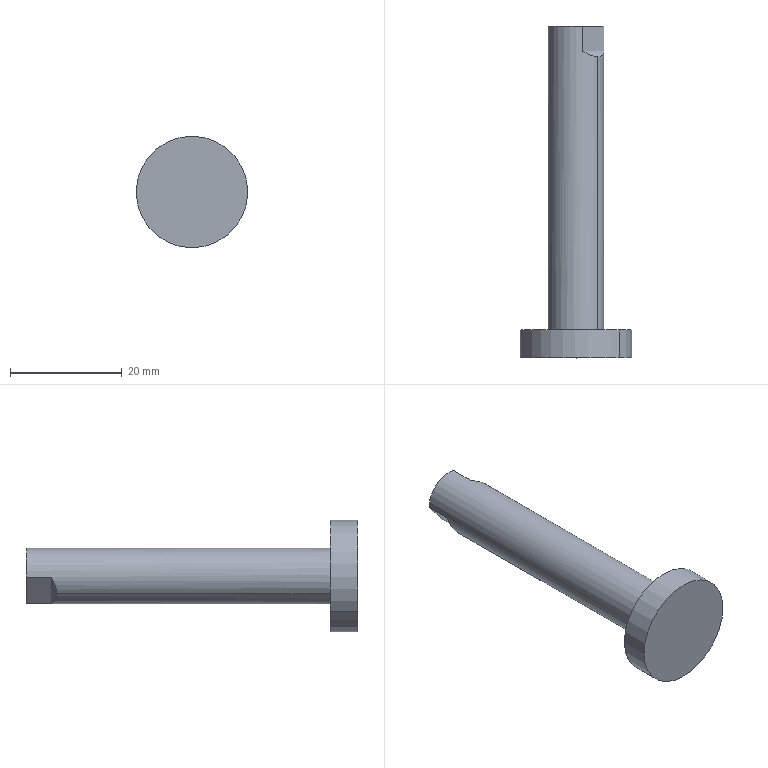Component | SolidWorks | BearingLiftingModule-1_CylinderLiftingModule-1_CDQ2B20-40DZ-L-M9B_0_0_0-1_CDQ2B20-40-M9B(0_0)_CYROD-1 | 1 solid | 17 faces | box 20 x 59.5 x 20 mm | volume 5711 mm3 | plane 7 | cylinder 6 | cone 4 | commonest cylinder face diameters 20 x2 10 x2 4.134 x2
STEP:
#1=COLOUR_RGB('',0.7922,0.8196,0.9333);
#2=FILL_AREA_STYLE_COLOUR('',#1);
#3=FILL_AREA_STYLE('',(#2));
#4=SURFACE_STYLE_FILL_AREA(#3);
#5=SURFACE_SIDE_STYLE('',(#4));
#6=SURFACE_STYLE_USAGE(.BOTH.,#5);
#7=PRESENTATION_STYLE_ASSIGNMENT((#6));
#8=CARTESIAN_POINT('',(2.451,-4.181,0.9322));
#9=VERTEX_POINT('',#8);
#10=CARTESIAN_POINT('',(3.061,-4.181,1.43));
#11=VERTEX_POINT('',#10);
#12=CARTESIAN_POINT('',(2.756,-4.181,1.181));
#13=DIRECTION('',(-0.,-1.,0.));
#14=DIRECTION('',(0.7749,0.,0.6321));
#15=AXIS2_PLACEMENT_3D('',#12,#13,#14);
#16=CIRCLE('',#15,0.3937);
#17=EDGE_CURVE('',#9,#11,#16,.T.);
#18=ORIENTED_EDGE('',*,*,#17,.F.);
#19=CARTESIAN_POINT('',(2.451,-3.984,0.9322));
#20=VERTEX_POINT('',#19);
#21=CARTESIAN_POINT('',(2.451,-4.181,0.9322));
#22=DIRECTION('',(0.,1.,-0.));
#23=VECTOR('',#22,39.37);
#24=LINE('',#21,#23);
#25=EDGE_CURVE('',#9,#20,#24,.T.);
#26=ORIENTED_EDGE('',*,*,#25,.T.);
#27=CARTESIAN_POINT('',(3.061,-3.984,1.43));
#28=VERTEX_POINT('',#27);
#29=CARTESIAN_POINT('',(2.756,-3.984,1.181));
#30=DIRECTION('',(-0.,-1.,0.));
#31=DIRECTION('',(0.7749,0.,0.6321));
#32=AXIS2_PLACEMENT_3D('',#29,#30,#31);
#33=CIRCLE('',#32,0.3937);
#34=EDGE_CURVE('',#20,#28,#33,.T.);
#35=ORIENTED_EDGE('',*,*,#34,.T.);
#36=CARTESIAN_POINT('',(3.061,-4.181,1.43));
#37=DIRECTION('',(0.,1.,-0.));
#38=VECTOR('',#37,39.37);
#39=LINE('',#36,#38);
#40=EDGE_CURVE('',#11,#28,#39,.T.);
#41=ORIENTED_EDGE('',*,*,#40,.F.);
#42=EDGE_LOOP('',(#18,#26,#35,#41));
#43=FACE_OUTER_BOUND('',#42,.T.);
#44=CARTESIAN_POINT('',(2.756,-4.181,1.181));
#45=DIRECTION('',(0.,1.,-0.));
#46=DIRECTION('',(0.7749,0.,0.6321));
#47=AXIS2_PLACEMENT_3D('',#44,#45,#46);
#48=CYLINDRICAL_SURFACE('',#47,0.3937);
#49=ADVANCED_FACE('',(#43),#48,.T.);
#50=CARTESIAN_POINT('',(2.693,-1.856,1.13));
#51=VERTEX_POINT('',#50);
#52=CARTESIAN_POINT('',(2.819,-1.856,1.233));
#53=VERTEX_POINT('',#52);
#54=CARTESIAN_POINT('',(2.756,-1.856,1.181));
#55=DIRECTION('',(-0.,-1.,0.));
#56=DIRECTION('',(0.7749,0.,0.6321));
#57=AXIS2_PLACEMENT_3D('',#54,#55,#56);
#58=CIRCLE('',#57,0.08138);
#59=EDGE_CURVE('',#51,#53,#58,.T.);
#60=ORIENTED_EDGE('',*,*,#59,.T.);
#61=CARTESIAN_POINT('',(2.832,-1.839,1.243));
#62=VERTEX_POINT('',#61);
#63=CARTESIAN_POINT('',(2.819,-1.856,1.233));
#64=DIRECTION('',(0.5479,0.7071,0.447));
#65=VECTOR('',#64,39.37);
#66=LINE('',#63,#65);
#67=EDGE_CURVE('',#53,#62,#66,.T.);
#68=ORIENTED_EDGE('',*,*,#67,.T.);
#69=CARTESIAN_POINT('',(2.68,-1.839,1.119));
#70=VERTEX_POINT('',#69);
#71=CARTESIAN_POINT('',(2.756,-1.839,1.181));
#72=DIRECTION('',(-0.,-1.,0.));
#73=DIRECTION('',(0.7749,0.,0.6321));
#74=AXIS2_PLACEMENT_3D('',#71,#72,#73);
#75=CIRCLE('',#74,0.09843);
#76=EDGE_CURVE('',#70,#62,#75,.T.);
#77=ORIENTED_EDGE('',*,*,#76,.F.);
#78=CARTESIAN_POINT('',(2.693,-1.856,1.13));
#79=DIRECTION('',(-0.5479,0.7071,-0.447));
#80=VECTOR('',#79,39.37);
#81=LINE('',#78,#80);
#82=EDGE_CURVE('',#51,#70,#81,.T.);
#83=ORIENTED_EDGE('',*,*,#82,.F.);
#84=EDGE_LOOP('',(#60,#68,#77,#83));
#85=FACE_OUTER_BOUND('',#84,.T.);
#86=CARTESIAN_POINT('',(2.756,-1.856,1.181));
#87=DIRECTION('',(0.,1.,-0.));
#88=DIRECTION('',(-0.7749,0.,-0.6321));
#89=AXIS2_PLACEMENT_3D('',#86,#87,#88);
#90=CONICAL_SURFACE('',#89,0.08138,0.7854);
#91=ADVANCED_FACE('',(#85),#90,.F.);
#92=CARTESIAN_POINT('',(2.603,-3.984,1.057));
#93=VERTEX_POINT('',#92);
#94=CARTESIAN_POINT('',(2.908,-3.984,1.306));
#95=VERTEX_POINT('',#94);
#96=CARTESIAN_POINT('',(2.756,-3.984,1.181));
#97=DIRECTION('',(-0.,-1.,0.));
#98=DIRECTION('',(0.7749,0.,0.6321));
#99=AXIS2_PLACEMENT_3D('',#96,#97,#98);
#100=CIRCLE('',#99,0.1969);
#101=EDGE_CURVE('',#93,#95,#100,.T.);
#102=ORIENTED_EDGE('',*,*,#101,.F.);
#103=CARTESIAN_POINT('',(2.603,-2.055,1.057));
#104=VERTEX_POINT('',#103);
#105=CARTESIAN_POINT('',(2.603,-4.181,1.057));
#106=DIRECTION('',(0.,1.,-0.));
#107=VECTOR('',#106,39.37);
#108=LINE('',#105,#107);
#109=EDGE_CURVE('',#93,#104,#108,.T.);
#110=ORIENTED_EDGE('',*,*,#109,.T.);
#111=CARTESIAN_POINT('',(2.709,-2.016,0.99));
#112=VERTEX_POINT('',#111);
#113=CARTESIAN_POINT('',(2.709,-2.016,0.99));
#114=CARTESIAN_POINT('',(2.667,-2.041,1.));
#115=CARTESIAN_POINT('',(2.631,-2.055,1.023));
#116=CARTESIAN_POINT('',(2.603,-2.055,1.057));
#117=(BOUNDED_CURVE()B_SPLINE_CURVE(3,(#113,#114,#115,#116),.UNSPECIFIED.,.F.,.F.)B_SPLINE_CURVE_WITH_KNOTS((4,4),(5.64,6.283),.UNSPECIFIED.)CURVE()GEOMETRIC_REPRESENTATION_ITEM()RATIONAL_B_SPLINE_CURVE((1.,0.9658,0.9658,1.))REPRESENTATION_ITEM(''));
#118=EDGE_CURVE('',#112,#104,#117,.T.);
#119=ORIENTED_EDGE('',*,*,#118,.F.);
#120=CARTESIAN_POINT('',(2.709,-1.839,0.99));
#121=VERTEX_POINT('',#120);
#122=CARTESIAN_POINT('',(2.709,-4.181,0.99));
#123=DIRECTION('',(-0.,-1.,0.));
#124=VECTOR('',#123,39.37);
#125=LINE('',#122,#124);
#126=EDGE_CURVE('',#121,#112,#125,.T.);
#127=ORIENTED_EDGE('',*,*,#126,.F.);
#128=CARTESIAN_POINT('',(2.953,-1.839,1.189));
#129=VERTEX_POINT('',#128);
#130=CARTESIAN_POINT('',(2.756,-1.839,1.181));
#131=DIRECTION('',(-0.,-1.,0.));
#132=DIRECTION('',(0.7749,0.,0.6321));
#133=AXIS2_PLACEMENT_3D('',#130,#131,#132);
#134=CIRCLE('',#133,0.1969);
#135=EDGE_CURVE('',#121,#129,#134,.T.);
#136=ORIENTED_EDGE('',*,*,#135,.T.);
#137=CARTESIAN_POINT('',(2.953,-2.016,1.189));
#138=VERTEX_POINT('',#137);
#139=CARTESIAN_POINT('',(2.953,-4.181,1.189));
#140=DIRECTION('',(0.,1.,-0.));
#141=VECTOR('',#140,39.37);
#142=LINE('',#139,#141);
#143=EDGE_CURVE('',#138,#129,#142,.T.);
#144=ORIENTED_EDGE('',*,*,#143,.F.);
#145=CARTESIAN_POINT('',(2.908,-2.055,1.306));
#146=VERTEX_POINT('',#145);
#147=CARTESIAN_POINT('',(2.908,-2.055,1.306));
#148=CARTESIAN_POINT('',(2.936,-2.055,1.272));
#149=CARTESIAN_POINT('',(2.951,-2.041,1.232));
#150=CARTESIAN_POINT('',(2.953,-2.016,1.189));
#151=(BOUNDED_CURVE()B_SPLINE_CURVE(3,(#147,#148,#149,#150),.UNSPECIFIED.,.F.,.F.)B_SPLINE_CURVE_WITH_KNOTS((4,4),(0.,0.6435),.UNSPECIFIED.)CURVE()GEOMETRIC_REPRESENTATION_ITEM()RATIONAL_B_SPLINE_CURVE((1.,0.9658,0.9658,1.))REPRESENTATION_ITEM(''));
#152=EDGE_CURVE('',#146,#138,#151,.T.);
#153=ORIENTED_EDGE('',*,*,#152,.F.);
#154=CARTESIAN_POINT('',(2.908,-4.181,1.306));
#155=DIRECTION('',(0.,1.,-0.));
#156=VECTOR('',#155,39.37);
#157=LINE('',#154,#156);
#158=EDGE_CURVE('',#95,#146,#157,.T.);
#159=ORIENTED_EDGE('',*,*,#158,.F.);
#160=EDGE_LOOP('',(#102,#110,#119,#127,#136,#144,#153,#159));
#161=FACE_OUTER_BOUND('',#160,.T.);
#162=CARTESIAN_POINT('',(2.756,-4.181,1.181));
#163=DIRECTION('',(0.,1.,-0.));
#164=DIRECTION('',(0.7749,0.,0.6321));
#165=AXIS2_PLACEMENT_3D('',#162,#163,#164);
#166=CYLINDRICAL_SURFACE('',#165,0.1969);
#167=ADVANCED_FACE('',(#161),#166,.T.);
#168=CARTESIAN_POINT('',(2.819,-2.114,1.233));
#169=VERTEX_POINT('',#168);
#170=CARTESIAN_POINT('',(2.693,-2.114,1.13));
#171=VERTEX_POINT('',#170);
#172=CARTESIAN_POINT('',(2.756,-2.114,1.181));
#173=DIRECTION('',(-0.,-1.,0.));
#174=DIRECTION('',(0.7749,0.,0.6321));
#175=AXIS2_PLACEMENT_3D('',#172,#173,#174);
#176=CIRCLE('',#175,0.08138);
#177=EDGE_CURVE('',#169,#171,#176,.T.);
#178=ORIENTED_EDGE('',*,*,#177,.T.);
#179=CARTESIAN_POINT('',(2.693,-4.181,1.13));
#180=DIRECTION('',(0.,1.,-0.));
#181=VECTOR('',#180,39.37);
#182=LINE('',#179,#181);
#183=EDGE_CURVE('',#171,#51,#182,.T.);
#184=ORIENTED_EDGE('',*,*,#183,.T.);
#185=CARTESIAN_POINT('',(2.756,-1.856,1.181));
#186=DIRECTION('',(-0.,-1.,0.));
#187=DIRECTION('',(0.7749,0.,0.6321));
#188=AXIS2_PLACEMENT_3D('',#185,#186,#187);
#189=CIRCLE('',#188,0.08138);
#190=EDGE_CURVE('',#53,#51,#189,.T.);
#191=ORIENTED_EDGE('',*,*,#190,.F.);
#192=CARTESIAN_POINT('',(2.819,-4.181,1.233));
#193=DIRECTION('',(0.,1.,-0.));
#194=VECTOR('',#193,39.37);
#195=LINE('',#192,#194);
#196=EDGE_CURVE('',#169,#53,#195,.T.);
#197=ORIENTED_EDGE('',*,*,#196,.F.);
#198=EDGE_LOOP('',(#178,#184,#191,#197));
#199=FACE_OUTER_BOUND('',#198,.T.);
#200=CARTESIAN_POINT('',(2.756,-4.181,1.181));
#201=DIRECTION('',(0.,1.,-0.));
#202=DIRECTION('',(0.7749,0.,0.6321));
#203=AXIS2_PLACEMENT_3D('',#200,#201,#202);
#204=CYLINDRICAL_SURFACE('',#203,0.08138);
#205=ADVANCED_FACE('',(#199),#204,.F.);
#206=CARTESIAN_POINT('',(2.756,-2.161,1.181));
#207=VERTEX_POINT('',#206);
#208=CARTESIAN_POINT('',(-23.664,17.524,-20.37));
#209=DIRECTION('',(-0.6711,0.5,-0.5474));
#210=VECTOR('',#209,39.37);
#211=LINE('',#208,#210);
#212=EDGE_CURVE('',#207,#171,#211,.T.);
#213=ORIENTED_EDGE('',*,*,#212,.F.);
#214=CARTESIAN_POINT('',(29.176,17.524,22.733));
#215=DIRECTION('',(0.6711,0.5,0.5474));
#216=VECTOR('',#215,39.37);
#217=LINE('',#214,#216);
#218=EDGE_CURVE('',#207,#169,#217,.T.);
#219=ORIENTED_EDGE('',*,*,#218,.T.);
#220=CARTESIAN_POINT('',(2.756,-2.114,1.181));
#221=DIRECTION('',(-0.,-1.,0.));
#222=DIRECTION('',(0.7749,0.,0.6321));
#223=AXIS2_PLACEMENT_3D('',#220,#221,#222);
#224=CIRCLE('',#223,0.08138);
#225=EDGE_CURVE('',#171,#169,#224,.T.);
#226=ORIENTED_EDGE('',*,*,#225,.F.);
#227=EDGE_LOOP('',(#213,#219,#226));
#228=FACE_OUTER_BOUND('',#227,.T.);
#229=CARTESIAN_POINT('',(2.756,17.524,1.181));
#230=DIRECTION('',(0.,1.,-0.));
#231=DIRECTION('',(-0.7749,0.,-0.6321));
#232=AXIS2_PLACEMENT_3D('',#229,#230,#231);
#233=CONICAL_SURFACE('',#232,34.095,1.047);
#234=ADVANCED_FACE('',(#228),#233,.F.);
#235=ORIENTED_EDGE('',*,*,#218,.F.);
#236=ORIENTED_EDGE('',*,*,#212,.T.);
#237=ORIENTED_EDGE('',*,*,#177,.F.);
#238=EDGE_LOOP('',(#235,#236,#237));
#239=FACE_OUTER_BOUND('',#238,.T.);
#240=CARTESIAN_POINT('',(2.756,17.524,1.181));
#241=DIRECTION('',(0.,1.,-0.));
#242=DIRECTION('',(-0.7749,0.,-0.6321));
#243=AXIS2_PLACEMENT_3D('',#240,#241,#242);
#244=CONICAL_SURFACE('',#243,34.095,1.047);
#245=ADVANCED_FACE('',(#239),#244,.F.);
#246=ORIENTED_EDGE('',*,*,#183,.F.);
#247=ORIENTED_EDGE('',*,*,#225,.T.);
#248=ORIENTED_EDGE('',*,*,#196,.T.);
#249=ORIENTED_EDGE('',*,*,#59,.F.);
#250=EDGE_LOOP('',(#246,#247,#248,#249));
#251=FACE_OUTER_BOUND('',#250,.T.);
#252=CARTESIAN_POINT('',(2.756,-4.181,1.181));
#253=DIRECTION('',(0.,1.,-0.));
#254=DIRECTION('',(0.7749,0.,0.6321));
#255=AXIS2_PLACEMENT_3D('',#252,#253,#254);
#256=CYLINDRICAL_SURFACE('',#255,0.08138);
#257=ADVANCED_FACE('',(#251),#256,.F.);
#258=ORIENTED_EDGE('',*,*,#109,.F.);
#259=CARTESIAN_POINT('',(2.756,-3.984,1.181));
#260=DIRECTION('',(-0.,-1.,0.));
#261=DIRECTION('',(0.7749,0.,0.6321));
#262=AXIS2_PLACEMENT_3D('',#259,#260,#261);
#263=CIRCLE('',#262,0.1969);
#264=EDGE_CURVE('',#95,#93,#263,.T.);
#265=ORIENTED_EDGE('',*,*,#264,.F.);
#266=ORIENTED_EDGE('',*,*,#158,.T.);
#267=CARTESIAN_POINT('',(2.803,-2.016,1.372));
#268=VERTEX_POINT('',#267);
#269=CARTESIAN_POINT('',(2.803,-2.016,1.372));
#270=CARTESIAN_POINT('',(2.845,-2.041,1.362));
#271=CARTESIAN_POINT('',(2.881,-2.055,1.339));
#272=CARTESIAN_POINT('',(2.908,-2.055,1.306));
#273=(BOUNDED_CURVE()B_SPLINE_CURVE(3,(#269,#270,#271,#272),.UNSPECIFIED.,.F.,.F.)B_SPLINE_CURVE_WITH_KNOTS((4,4),(5.64,6.283),.UNSPECIFIED.)CURVE()GEOMETRIC_REPRESENTATION_ITEM()RATIONAL_B_SPLINE_CURVE((1.,0.9658,0.9658,1.))REPRESENTATION_ITEM(''));
#274=EDGE_CURVE('',#268,#146,#273,.T.);
#275=ORIENTED_EDGE('',*,*,#274,.F.);
#276=CARTESIAN_POINT('',(2.803,-1.839,1.372));
#277=VERTEX_POINT('',#276);
#278=CARTESIAN_POINT('',(2.803,-4.181,1.372));
#279=DIRECTION('',(-0.,-1.,0.));
#280=VECTOR('',#279,39.37);
#281=LINE('',#278,#280);
#282=EDGE_CURVE('',#277,#268,#281,.T.);
#283=ORIENTED_EDGE('',*,*,#282,.F.);
#284=CARTESIAN_POINT('',(2.559,-1.839,1.173));
#285=VERTEX_POINT('',#284);
#286=CARTESIAN_POINT('',(2.756,-1.839,1.181));
#287=DIRECTION('',(-0.,-1.,0.));
#288=DIRECTION('',(0.7749,0.,0.6321));
#289=AXIS2_PLACEMENT_3D('',#286,#287,#288);
#290=CIRCLE('',#289,0.1969);
#291=EDGE_CURVE('',#277,#285,#290,.T.);
#292=ORIENTED_EDGE('',*,*,#291,.T.);
#293=CARTESIAN_POINT('',(2.559,-2.016,1.173));
#294=VERTEX_POINT('',#293);
#295=CARTESIAN_POINT('',(2.559,-4.181,1.173));
#296=DIRECTION('',(0.,1.,-0.));
#297=VECTOR('',#296,39.37);
#298=LINE('',#295,#297);
#299=EDGE_CURVE('',#294,#285,#298,.T.);
#300=ORIENTED_EDGE('',*,*,#299,.F.);
#301=CARTESIAN_POINT('',(2.603,-2.055,1.057));
#302=CARTESIAN_POINT('',(2.576,-2.055,1.09));
#303=CARTESIAN_POINT('',(2.561,-2.041,1.13));
#304=CARTESIAN_POINT('',(2.559,-2.016,1.173));
#305=(BOUNDED_CURVE()B_SPLINE_CURVE(3,(#301,#302,#303,#304),.UNSPECIFIED.,.F.,.F.)B_SPLINE_CURVE_WITH_KNOTS((4,4),(0.,0.6435),.UNSPECIFIED.)CURVE()GEOMETRIC_REPRESENTATION_ITEM()RATIONAL_B_SPLINE_CURVE((1.,0.9658,0.9658,1.))REPRESENTATION_ITEM(''));
#306=EDGE_CURVE('',#104,#294,#305,.T.);
#307=ORIENTED_EDGE('',*,*,#306,.F.);
#308=EDGE_LOOP('',(#258,#265,#266,#275,#283,#292,#300,#307));
#309=FACE_OUTER_BOUND('',#308,.T.);
#310=CARTESIAN_POINT('',(2.756,-4.181,1.181));
#311=DIRECTION('',(0.,1.,-0.));
#312=DIRECTION('',(0.7749,0.,0.6321));
#313=AXIS2_PLACEMENT_3D('',#310,#311,#312);
#314=CYLINDRICAL_SURFACE('',#313,0.1969);
#315=ADVANCED_FACE('',(#309),#314,.T.);
#316=ORIENTED_EDGE('',*,*,#291,.F.);
#317=CARTESIAN_POINT('',(2.629,-1.839,1.586));
#318=DIRECTION('',(0.6321,-0.,-0.7749));
#319=VECTOR('',#318,39.37);
#320=LINE('',#317,#319);
#321=EDGE_CURVE('',#277,#129,#320,.T.);
#322=ORIENTED_EDGE('',*,*,#321,.T.);
#323=ORIENTED_EDGE('',*,*,#135,.F.);
#324=CARTESIAN_POINT('',(2.385,-1.839,1.387));
#325=DIRECTION('',(0.6321,-0.,-0.7749));
#326=VECTOR('',#325,39.37);
#327=LINE('',#324,#326);
#328=EDGE_CURVE('',#285,#121,#327,.T.);
#329=ORIENTED_EDGE('',*,*,#328,.F.);
#330=EDGE_LOOP('',(#316,#322,#323,#329));
#331=FACE_OUTER_BOUND('',#330,.T.);
#332=ORIENTED_EDGE('',*,*,#76,.T.);
#333=CARTESIAN_POINT('',(2.756,-1.839,1.181));
#334=DIRECTION('',(-0.,-1.,0.));
#335=DIRECTION('',(0.7749,0.,0.6321));
#336=AXIS2_PLACEMENT_3D('',#333,#334,#335);
#337=CIRCLE('',#336,0.09843);
#338=EDGE_CURVE('',#62,#70,#337,.T.);
#339=ORIENTED_EDGE('',*,*,#338,.T.);
#340=EDGE_LOOP('',(#332,#339));
#341=FACE_BOUND('',#340,.T.);
#342=CARTESIAN_POINT('',(2.694,-1.839,1.257));
#343=DIRECTION('',(0.,-1.,0.));
#344=DIRECTION('',(-0.6321,0.,0.7749));
#345=AXIS2_PLACEMENT_3D('',#342,#343,#344);
#346=PLANE('',#345);
#347=ADVANCED_FACE('',(#331,#341),#346,.F.);
#348=ORIENTED_EDGE('',*,*,#67,.F.);
#349=ORIENTED_EDGE('',*,*,#190,.T.);
#350=ORIENTED_EDGE('',*,*,#82,.T.);
#351=ORIENTED_EDGE('',*,*,#338,.F.);
#352=EDGE_LOOP('',(#348,#349,#350,#351));
#353=FACE_OUTER_BOUND('',#352,.T.);
#354=CARTESIAN_POINT('',(2.756,-1.856,1.181));
#355=DIRECTION('',(0.,1.,-0.));
#356=DIRECTION('',(-0.7749,0.,-0.6321));
#357=AXIS2_PLACEMENT_3D('',#354,#355,#356);
#358=CONICAL_SURFACE('',#357,0.08138,0.7854);
#359=ADVANCED_FACE('',(#353),#358,.F.);
#360=CARTESIAN_POINT('',(2.756,-3.984,1.181));
#361=DIRECTION('',(-0.,-1.,0.));
#362=DIRECTION('',(0.7749,0.,0.6321));
#363=AXIS2_PLACEMENT_3D('',#360,#361,#362);
#364=CIRCLE('',#363,0.3937);
#365=EDGE_CURVE('',#28,#20,#364,.T.);
#366=ORIENTED_EDGE('',*,*,#365,.F.);
#367=ORIENTED_EDGE('',*,*,#34,.F.);
#368=EDGE_LOOP('',(#366,#367));
#369=FACE_OUTER_BOUND('',#368,.T.);
#370=ORIENTED_EDGE('',*,*,#264,.T.);
#371=ORIENTED_EDGE('',*,*,#101,.T.);
#372=EDGE_LOOP('',(#370,#371));
#373=FACE_BOUND('',#372,.T.);
#374=CARTESIAN_POINT('',(2.631,-3.984,1.334));
#375=DIRECTION('',(0.,-1.,0.));
#376=DIRECTION('',(-0.6321,0.,0.7749));
#377=AXIS2_PLACEMENT_3D('',#374,#375,#376);
#378=PLANE('',#377);
#379=ADVANCED_FACE('',(#369,#373),#378,.F.);
#380=ORIENTED_EDGE('',*,*,#25,.F.);
#381=CARTESIAN_POINT('',(2.756,-4.181,1.181));
#382=DIRECTION('',(-0.,-1.,0.));
#383=DIRECTION('',(0.7749,0.,0.6321));
#384=AXIS2_PLACEMENT_3D('',#381,#382,#383);
#385=CIRCLE('',#384,0.3937);
#386=EDGE_CURVE('',#11,#9,#385,.T.);
#387=ORIENTED_EDGE('',*,*,#386,.F.);
#388=ORIENTED_EDGE('',*,*,#40,.T.);
#389=ORIENTED_EDGE('',*,*,#365,.T.);
#390=EDGE_LOOP('',(#380,#387,#388,#389));
#391=FACE_OUTER_BOUND('',#390,.T.);
#392=CARTESIAN_POINT('',(2.756,-4.181,1.181));
#393=DIRECTION('',(0.,1.,-0.));
#394=DIRECTION('',(0.7749,0.,0.6321));
#395=AXIS2_PLACEMENT_3D('',#392,#393,#394);
#396=CYLINDRICAL_SURFACE('',#395,0.3937);
#397=ADVANCED_FACE('',(#391),#396,.T.);
#398=ORIENTED_EDGE('',*,*,#386,.T.);
#399=ORIENTED_EDGE('',*,*,#17,.T.);
#400=EDGE_LOOP('',(#398,#399));
#401=FACE_OUTER_BOUND('',#400,.T.);
#402=CARTESIAN_POINT('',(2.507,-4.181,1.486));
#403=DIRECTION('',(-0.,1.,-0.));
#404=DIRECTION('',(-0.7749,-0.,-0.6321));
#405=AXIS2_PLACEMENT_3D('',#402,#403,#404);
#406=PLANE('',#405);
#407=ADVANCED_FACE('',(#401),#406,.F.);
#408=ORIENTED_EDGE('',*,*,#118,.T.);
#409=ORIENTED_EDGE('',*,*,#306,.T.);
#410=CARTESIAN_POINT('',(2.385,-2.016,1.387));
#411=DIRECTION('',(0.6321,-0.,-0.7749));
#412=VECTOR('',#411,39.37);
#413=LINE('',#410,#412);
#414=EDGE_CURVE('',#294,#112,#413,.T.);
#415=ORIENTED_EDGE('',*,*,#414,.T.);
#416=EDGE_LOOP('',(#408,#409,#415));
#417=FACE_OUTER_BOUND('',#416,.T.);
#418=CARTESIAN_POINT('',(2.232,-2.213,1.262));
#419=DIRECTION('',(-0.5479,0.7071,-0.447));
#420=DIRECTION('',(-0.6321,0.,0.7749));
#421=AXIS2_PLACEMENT_3D('',#418,#419,#420);
#422=PLANE('',#421);
#423=ADVANCED_FACE('',(#417),#422,.T.);
#424=ORIENTED_EDGE('',*,*,#126,.T.);
#425=ORIENTED_EDGE('',*,*,#414,.F.);
#426=ORIENTED_EDGE('',*,*,#299,.T.);
#427=ORIENTED_EDGE('',*,*,#328,.T.);
#428=EDGE_LOOP('',(#424,#425,#426,#427));
#429=FACE_OUTER_BOUND('',#428,.T.);
#430=CARTESIAN_POINT('',(2.385,-2.016,1.387));
#431=DIRECTION('',(-0.7749,-0.,-0.6321));
#432=DIRECTION('',(-0.,-1.,0.));
#433=AXIS2_PLACEMENT_3D('',#430,#431,#432);
#434=PLANE('',#433);
#435=ADVANCED_FACE('',(#429),#434,.T.);
#436=ORIENTED_EDGE('',*,*,#282,.T.);
#437=CARTESIAN_POINT('',(2.629,-2.016,1.586));
#438=DIRECTION('',(0.6321,-0.,-0.7749));
#439=VECTOR('',#438,39.37);
#440=LINE('',#437,#439);
#441=EDGE_CURVE('',#268,#138,#440,.T.);
#442=ORIENTED_EDGE('',*,*,#441,.T.);
#443=ORIENTED_EDGE('',*,*,#143,.T.);
#444=ORIENTED_EDGE('',*,*,#321,.F.);
#445=EDGE_LOOP('',(#436,#442,#443,#444));
#446=FACE_OUTER_BOUND('',#445,.T.);
#447=CARTESIAN_POINT('',(2.629,-1.839,1.586));
#448=DIRECTION('',(0.7749,0.,0.6321));
#449=DIRECTION('',(0.6321,-0.,-0.7749));
#450=AXIS2_PLACEMENT_3D('',#447,#448,#449);
#451=PLANE('',#450);
#452=ADVANCED_FACE('',(#446),#451,.T.);
#453=ORIENTED_EDGE('',*,*,#274,.T.);
#454=ORIENTED_EDGE('',*,*,#152,.T.);
#455=ORIENTED_EDGE('',*,*,#441,.F.);
#456=EDGE_LOOP('',(#453,#454,#455));
#457=FACE_OUTER_BOUND('',#456,.T.);
#458=CARTESIAN_POINT('',(2.629,-2.016,1.586));
#459=DIRECTION('',(0.5479,0.7071,0.447));
#460=DIRECTION('',(-0.5479,0.7071,-0.447));
#461=AXIS2_PLACEMENT_3D('',#458,#459,#460);
#462=PLANE('',#461);
#463=ADVANCED_FACE('',(#457),#462,.T.);
#464=CLOSED_SHELL('',(#49,#91,#167,#205,#234,#245,#257,#315,#347,#359,#379,#397,#407,#423,#435,#452,#463));
#465=MANIFOLD_SOLID_BREP('',#464);
#466=STYLED_ITEM('',(#7),#465);
#467=(LENGTH_UNIT()NAMED_UNIT(*)SI_UNIT($,.METRE.));
#468=LENGTH_MEASURE_WITH_UNIT(LENGTH_MEASURE(0.0254),#467);
#469=DIMENSIONAL_EXPONENTS(1.,0.,0.,0.,0.,0.,0.);
#470=(CONVERSION_BASED_UNIT('',#468)LENGTH_UNIT()NAMED_UNIT(#469));
#471=UNCERTAINTY_MEASURE_WITH_UNIT(LENGTH_MEASURE(0.00001),#470,'','');
#472=(NAMED_UNIT(*)PLANE_ANGLE_UNIT()SI_UNIT($,.RADIAN.));
#473=(NAMED_UNIT(*)SI_UNIT($,.STERADIAN.)SOLID_ANGLE_UNIT());
#474=(GEOMETRIC_REPRESENTATION_CONTEXT(3)GLOBAL_UNCERTAINTY_ASSIGNED_CONTEXT((#471))GLOBAL_UNIT_ASSIGNED_CONTEXT((#470,#472,#473))REPRESENTATION_CONTEXT('',''));
#475=MECHANICAL_DESIGN_GEOMETRIC_PRESENTATION_REPRESENTATION('',(#466),#474);
#476=PRESENTATION_LAYER_ASSIGNMENT('','',(#466));
#477=CARTESIAN_POINT('',(0.,0.,0.));
#478=DIRECTION('',(0.,0.,1.));
#479=DIRECTION('',(1.,0.,0.));
#480=AXIS2_PLACEMENT_3D('',#477,#478,#479);
#481=(LENGTH_UNIT()NAMED_UNIT(*)SI_UNIT($,.METRE.));
#482=LENGTH_MEASURE_WITH_UNIT(LENGTH_MEASURE(0.0254),#481);
#483=DIMENSIONAL_EXPONENTS(1.,0.,0.,0.,0.,0.,0.);
#484=(CONVERSION_BASED_UNIT('',#482)LENGTH_UNIT()NAMED_UNIT(#483));
#485=UNCERTAINTY_MEASURE_WITH_UNIT(LENGTH_MEASURE(0.00001),#484,'','');
#486=(NAMED_UNIT(*)PLANE_ANGLE_UNIT()SI_UNIT($,.RADIAN.));
#487=(NAMED_UNIT(*)SI_UNIT($,.STERADIAN.)SOLID_ANGLE_UNIT());
#488=(GEOMETRIC_REPRESENTATION_CONTEXT(3)GLOBAL_UNCERTAINTY_ASSIGNED_CONTEXT((#485))GLOBAL_UNIT_ASSIGNED_CONTEXT((#484,#486,#487))REPRESENTATION_CONTEXT('',''));
#489=ADVANCED_BREP_SHAPE_REPRESENTATION('',(#465,#480),#488);